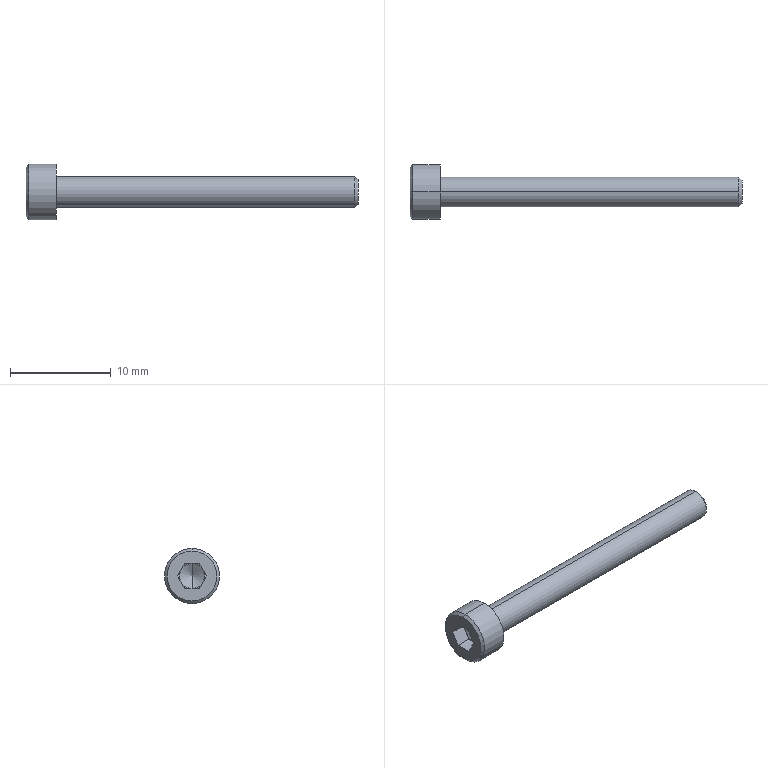Component | SolidWorks | TAC21-M3-L30Screw-1 | 1 solid | 25 faces | box 33 x 5.5 x 5.5 mm | volume 273 mm3 | plane 15 | cone 6 | cylinder 4 | commonest cylinder face diameters 3 x2 5.5 x2
STEP:
#1=COLOUR_RGB('',0.7922,0.8196,0.9333);
#2=FILL_AREA_STYLE_COLOUR('',#1);
#3=FILL_AREA_STYLE('',(#2));
#4=SURFACE_STYLE_FILL_AREA(#3);
#5=SURFACE_SIDE_STYLE('',(#4));
#6=SURFACE_STYLE_USAGE(.BOTH.,#5);
#7=PRESENTATION_STYLE_ASSIGNMENT((#6));
#8=CARTESIAN_POINT('',(-4.015,0.6298,4.665));
#9=VERTEX_POINT('',#8);
#10=CARTESIAN_POINT('',(-4.015,0.6298,4.547));
#11=VERTEX_POINT('',#10);
#12=CARTESIAN_POINT('',(-4.015,0.6298,4.606));
#13=DIRECTION('',(-1.,0.,0.));
#14=DIRECTION('',(0.,0.,1.));
#15=AXIS2_PLACEMENT_3D('',#12,#13,#14);
#16=CIRCLE('',#15,0.05906);
#17=EDGE_CURVE('',#9,#11,#16,.T.);
#18=ORIENTED_EDGE('',*,*,#17,.T.);
#19=CARTESIAN_POINT('',(-5.184,0.6298,4.547));
#20=VERTEX_POINT('',#19);
#21=CARTESIAN_POINT('',(-4.002,0.6298,4.547));
#22=DIRECTION('',(-1.,0.,0.));
#23=VECTOR('',#22,39.37);
#24=LINE('',#21,#23);
#25=EDGE_CURVE('',#11,#20,#24,.T.);
#26=ORIENTED_EDGE('',*,*,#25,.T.);
#27=CARTESIAN_POINT('',(-5.184,0.6298,4.665));
#28=VERTEX_POINT('',#27);
#29=CARTESIAN_POINT('',(-5.184,0.6298,4.606));
#30=DIRECTION('',(1.,0.,-0.));
#31=DIRECTION('',(0.,0.,1.));
#32=AXIS2_PLACEMENT_3D('',#29,#30,#31);
#33=CIRCLE('',#32,0.05906);
#34=EDGE_CURVE('',#20,#28,#33,.T.);
#35=ORIENTED_EDGE('',*,*,#34,.T.);
#36=CARTESIAN_POINT('',(-4.002,0.6298,4.665));
#37=DIRECTION('',(-1.,0.,0.));
#38=VECTOR('',#37,39.37);
#39=LINE('',#36,#38);
#40=EDGE_CURVE('',#9,#28,#39,.T.);
#41=ORIENTED_EDGE('',*,*,#40,.F.);
#42=EDGE_LOOP('',(#18,#26,#35,#41));
#43=FACE_OUTER_BOUND('',#42,.T.);
#44=CARTESIAN_POINT('',(-4.002,0.6298,4.606));
#45=DIRECTION('',(-1.,0.,0.));
#46=DIRECTION('',(0.,0.,1.));
#47=AXIS2_PLACEMENT_3D('',#44,#45,#46);
#48=CYLINDRICAL_SURFACE('',#47,0.05906);
#49=ADVANCED_FACE('',(#43),#48,.T.);
#50=CARTESIAN_POINT('',(-4.002,0.6298,4.653));
#51=VERTEX_POINT('',#50);
#52=CARTESIAN_POINT('',(-4.002,0.6298,4.559));
#53=VERTEX_POINT('',#52);
#54=CARTESIAN_POINT('',(-4.002,0.6298,4.606));
#55=DIRECTION('',(-1.,0.,0.));
#56=DIRECTION('',(0.,0.,1.));
#57=AXIS2_PLACEMENT_3D('',#54,#55,#56);
#58=CIRCLE('',#57,0.04699);
#59=EDGE_CURVE('',#51,#53,#58,.T.);
#60=ORIENTED_EDGE('',*,*,#59,.T.);
#61=CARTESIAN_POINT('',(-4.015,0.6298,4.547));
#62=DIRECTION('',(-0.7071,0.,-0.7071));
#63=VECTOR('',#62,39.37);
#64=LINE('',#61,#63);
#65=EDGE_CURVE('',#53,#11,#64,.T.);
#66=ORIENTED_EDGE('',*,*,#65,.T.);
#67=ORIENTED_EDGE('',*,*,#17,.F.);
#68=CARTESIAN_POINT('',(-4.015,0.6298,4.665));
#69=DIRECTION('',(-0.7071,0.,0.7071));
#70=VECTOR('',#69,39.37);
#71=LINE('',#68,#70);
#72=EDGE_CURVE('',#51,#9,#71,.T.);
#73=ORIENTED_EDGE('',*,*,#72,.F.);
#74=EDGE_LOOP('',(#60,#66,#67,#73));
#75=FACE_OUTER_BOUND('',#74,.T.);
#76=CARTESIAN_POINT('',(-4.015,0.6298,4.606));
#77=DIRECTION('',(-1.,0.,0.));
#78=DIRECTION('',(0.,0.,1.));
#79=AXIS2_PLACEMENT_3D('',#76,#77,#78);
#80=CONICAL_SURFACE('',#79,0.05906,0.7854);
#81=ADVANCED_FACE('',(#75),#80,.T.);
#82=CARTESIAN_POINT('',(-5.184,0.6298,4.715));
#83=VERTEX_POINT('',#82);
#84=CARTESIAN_POINT('',(-5.184,0.6298,4.498));
#85=VERTEX_POINT('',#84);
#86=CARTESIAN_POINT('',(-5.184,0.6298,4.606));
#87=DIRECTION('',(-1.,0.,0.));
#88=DIRECTION('',(0.,0.,1.));
#89=AXIS2_PLACEMENT_3D('',#86,#87,#88);
#90=CIRCLE('',#89,0.1083);
#91=EDGE_CURVE('',#83,#85,#90,.T.);
#92=ORIENTED_EDGE('',*,*,#91,.T.);
#93=CARTESIAN_POINT('',(-5.291,0.6298,4.498));
#94=VERTEX_POINT('',#93);
#95=CARTESIAN_POINT('',(-5.184,0.6298,4.498));
#96=DIRECTION('',(-1.,0.,0.));
#97=VECTOR('',#96,39.37);
#98=LINE('',#95,#97);
#99=EDGE_CURVE('',#85,#94,#98,.T.);
#100=ORIENTED_EDGE('',*,*,#99,.T.);
#101=CARTESIAN_POINT('',(-5.291,0.6298,4.715));
#102=VERTEX_POINT('',#101);
#103=CARTESIAN_POINT('',(-5.291,0.6298,4.606));
#104=DIRECTION('',(1.,0.,-0.));
#105=DIRECTION('',(0.,0.,1.));
#106=AXIS2_PLACEMENT_3D('',#103,#104,#105);
#107=CIRCLE('',#106,0.1083);
#108=EDGE_CURVE('',#94,#102,#107,.T.);
#109=ORIENTED_EDGE('',*,*,#108,.T.);
#110=CARTESIAN_POINT('',(-5.184,0.6298,4.715));
#111=DIRECTION('',(-1.,0.,0.));
#112=VECTOR('',#111,39.37);
#113=LINE('',#110,#112);
#114=EDGE_CURVE('',#83,#102,#113,.T.);
#115=ORIENTED_EDGE('',*,*,#114,.F.);
#116=EDGE_LOOP('',(#92,#100,#109,#115));
#117=FACE_OUTER_BOUND('',#116,.T.);
#118=CARTESIAN_POINT('',(-5.184,0.6298,4.606));
#119=DIRECTION('',(-1.,0.,0.));
#120=DIRECTION('',(0.,0.,1.));
#121=AXIS2_PLACEMENT_3D('',#118,#119,#120);
#122=CYLINDRICAL_SURFACE('',#121,0.1083);
#123=ADVANCED_FACE('',(#117),#122,.T.);
#124=CARTESIAN_POINT('',(-5.302,0.6298,4.509));
#125=VERTEX_POINT('',#124);
#126=CARTESIAN_POINT('',(-5.302,0.6298,4.704));
#127=VERTEX_POINT('',#126);
#128=CARTESIAN_POINT('',(-5.302,0.6298,4.606));
#129=DIRECTION('',(1.,0.,-0.));
#130=DIRECTION('',(0.,0.,-1.));
#131=AXIS2_PLACEMENT_3D('',#128,#129,#130);
#132=CIRCLE('',#131,0.09744);
#133=EDGE_CURVE('',#125,#127,#132,.T.);
#134=ORIENTED_EDGE('',*,*,#133,.T.);
#135=CARTESIAN_POINT('',(-5.291,0.6298,4.715));
#136=DIRECTION('',(0.7071,0.,0.7071));
#137=VECTOR('',#136,39.37);
#138=LINE('',#135,#137);
#139=EDGE_CURVE('',#127,#102,#138,.T.);
#140=ORIENTED_EDGE('',*,*,#139,.T.);
#141=ORIENTED_EDGE('',*,*,#108,.F.);
#142=CARTESIAN_POINT('',(-5.291,0.6298,4.498));
#143=DIRECTION('',(0.7071,0.,-0.7071));
#144=VECTOR('',#143,39.37);
#145=LINE('',#142,#144);
#146=EDGE_CURVE('',#125,#94,#145,.T.);
#147=ORIENTED_EDGE('',*,*,#146,.F.);
#148=EDGE_LOOP('',(#134,#140,#141,#147));
#149=FACE_OUTER_BOUND('',#148,.T.);
#150=CARTESIAN_POINT('',(-5.291,0.6298,4.606));
#151=DIRECTION('',(1.,0.,-0.));
#152=DIRECTION('',(0.,0.,-1.));
#153=AXIS2_PLACEMENT_3D('',#150,#151,#152);
#154=CONICAL_SURFACE('',#153,0.1083,0.7854);
#155=ADVANCED_FACE('',(#149),#154,.T.);
#156=CARTESIAN_POINT('',(-5.214,0.6298,4.606));
#157=VERTEX_POINT('',#156);
#158=CARTESIAN_POINT('',(-5.243,0.6298,4.656));
#159=VERTEX_POINT('',#158);
#160=CARTESIAN_POINT('',(-5.243,0.6298,4.656));
#161=DIRECTION('',(-0.5,0.,0.866));
#162=VECTOR('',#161,39.37);
#163=LINE('',#160,#162);
#164=EDGE_CURVE('',#157,#159,#163,.T.);
#165=ORIENTED_EDGE('',*,*,#164,.F.);
#166=CARTESIAN_POINT('',(-5.243,0.6298,4.557));
#167=VERTEX_POINT('',#166);
#168=CARTESIAN_POINT('',(-5.243,0.6298,4.557));
#169=DIRECTION('',(-0.5,0.,-0.866));
#170=VECTOR('',#169,39.37);
#171=LINE('',#168,#170);
#172=EDGE_CURVE('',#157,#167,#171,.T.);
#173=ORIENTED_EDGE('',*,*,#172,.T.);
#174=CARTESIAN_POINT('',(-5.243,0.5871,4.582));
#175=VERTEX_POINT('',#174);
#176=CARTESIAN_POINT('',(-5.243,0.6298,4.606));
#177=DIRECTION('',(1.,0.,-0.));
#178=DIRECTION('',(0.,0.,1.));
#179=AXIS2_PLACEMENT_3D('',#176,#177,#178);
#180=CIRCLE('',#179,0.04921);
#181=EDGE_CURVE('',#175,#167,#180,.T.);
#182=ORIENTED_EDGE('',*,*,#181,.F.);
#183=CARTESIAN_POINT('',(-5.243,0.5871,4.631));
#184=VERTEX_POINT('',#183);
#185=CARTESIAN_POINT('',(-5.243,0.6298,4.606));
#186=DIRECTION('',(1.,0.,-0.));
#187=DIRECTION('',(0.,-0.,1.));
#188=AXIS2_PLACEMENT_3D('',#185,#186,#187);
#189=CIRCLE('',#188,0.04921);
#190=EDGE_CURVE('',#184,#175,#189,.T.);
#191=ORIENTED_EDGE('',*,*,#190,.F.);
#192=CARTESIAN_POINT('',(-5.243,0.6298,4.606));
#193=DIRECTION('',(1.,0.,-0.));
#194=DIRECTION('',(0.,0.,1.));
#195=AXIS2_PLACEMENT_3D('',#192,#193,#194);
#196=CIRCLE('',#195,0.04921);
#197=EDGE_CURVE('',#159,#184,#196,.T.);
#198=ORIENTED_EDGE('',*,*,#197,.F.);
#199=EDGE_LOOP('',(#165,#173,#182,#191,#198));
#200=FACE_OUTER_BOUND('',#199,.T.);
#201=CARTESIAN_POINT('',(-5.243,0.6298,4.606));
#202=DIRECTION('',(-1.,0.,0.));
#203=DIRECTION('',(0.,0.,1.));
#204=AXIS2_PLACEMENT_3D('',#201,#202,#203);
#205=CONICAL_SURFACE('',#204,0.04921,1.047);
#206=ADVANCED_FACE('',(#200),#205,.F.);
#207=ORIENTED_EDGE('',*,*,#25,.F.);
#208=CARTESIAN_POINT('',(-4.015,0.6298,4.606));
#209=DIRECTION('',(-1.,0.,0.));
#210=DIRECTION('',(0.,0.,1.));
#211=AXIS2_PLACEMENT_3D('',#208,#209,#210);
#212=CIRCLE('',#211,0.05906);
#213=EDGE_CURVE('',#11,#9,#212,.T.);
#214=ORIENTED_EDGE('',*,*,#213,.T.);
#215=ORIENTED_EDGE('',*,*,#40,.T.);
#216=CARTESIAN_POINT('',(-5.184,0.6298,4.606));
#217=DIRECTION('',(1.,0.,-0.));
#218=DIRECTION('',(0.,0.,1.));
#219=AXIS2_PLACEMENT_3D('',#216,#217,#218);
#220=CIRCLE('',#219,0.05906);
#221=EDGE_CURVE('',#28,#20,#220,.T.);
#222=ORIENTED_EDGE('',*,*,#221,.T.);
#223=EDGE_LOOP('',(#207,#214,#215,#222));
#224=FACE_OUTER_BOUND('',#223,.T.);
#225=CARTESIAN_POINT('',(-4.002,0.6298,4.606));
#226=DIRECTION('',(-1.,0.,0.));
#227=DIRECTION('',(0.,0.,1.));
#228=AXIS2_PLACEMENT_3D('',#225,#226,#227);
#229=CYLINDRICAL_SURFACE('',#228,0.05906);
#230=ADVANCED_FACE('',(#224),#229,.T.);
#231=ORIENTED_EDGE('',*,*,#91,.F.);
#232=CARTESIAN_POINT('',(-5.184,0.6298,4.606));
#233=DIRECTION('',(-1.,0.,0.));
#234=DIRECTION('',(0.,0.,1.));
#235=AXIS2_PLACEMENT_3D('',#232,#233,#234);
#236=CIRCLE('',#235,0.1083);
#237=EDGE_CURVE('',#85,#83,#236,.T.);
#238=ORIENTED_EDGE('',*,*,#237,.F.);
#239=EDGE_LOOP('',(#231,#238));
#240=FACE_OUTER_BOUND('',#239,.T.);
#241=ORIENTED_EDGE('',*,*,#221,.F.);
#242=ORIENTED_EDGE('',*,*,#34,.F.);
#243=EDGE_LOOP('',(#241,#242));
#244=FACE_BOUND('',#243,.T.);
#245=CARTESIAN_POINT('',(-5.184,0.738,4.606));
#246=DIRECTION('',(-1.,0.,0.));
#247=DIRECTION('',(0.,0.,1.));
#248=AXIS2_PLACEMENT_3D('',#245,#246,#247);
#249=PLANE('',#248);
#250=ADVANCED_FACE('',(#240,#244),#249,.F.);
#251=ORIENTED_EDGE('',*,*,#65,.F.);
#252=CARTESIAN_POINT('',(-4.002,0.6298,4.606));
#253=DIRECTION('',(-1.,0.,0.));
#254=DIRECTION('',(0.,0.,1.));
#255=AXIS2_PLACEMENT_3D('',#252,#253,#254);
#256=CIRCLE('',#255,0.04699);
#257=EDGE_CURVE('',#53,#51,#256,.T.);
#258=ORIENTED_EDGE('',*,*,#257,.T.);
#259=ORIENTED_EDGE('',*,*,#72,.T.);
#260=ORIENTED_EDGE('',*,*,#213,.F.);
#261=EDGE_LOOP('',(#251,#258,#259,#260));
#262=FACE_OUTER_BOUND('',#261,.T.);
#263=CARTESIAN_POINT('',(-4.015,0.6298,4.606));
#264=DIRECTION('',(-1.,0.,0.));
#265=DIRECTION('',(0.,0.,1.));
#266=AXIS2_PLACEMENT_3D('',#263,#264,#265);
#267=CONICAL_SURFACE('',#266,0.05906,0.7854);
#268=ADVANCED_FACE('',(#262),#267,.T.);
#269=ORIENTED_EDGE('',*,*,#99,.F.);
#270=ORIENTED_EDGE('',*,*,#237,.T.);
#271=ORIENTED_EDGE('',*,*,#114,.T.);
#272=CARTESIAN_POINT('',(-5.291,0.6298,4.606));
#273=DIRECTION('',(1.,0.,-0.));
#274=DIRECTION('',(0.,0.,1.));
#275=AXIS2_PLACEMENT_3D('',#272,#273,#274);
#276=CIRCLE('',#275,0.1083);
#277=EDGE_CURVE('',#102,#94,#276,.T.);
#278=ORIENTED_EDGE('',*,*,#277,.T.);
#279=EDGE_LOOP('',(#269,#270,#271,#278));
#280=FACE_OUTER_BOUND('',#279,.T.);
#281=CARTESIAN_POINT('',(-5.184,0.6298,4.606));
#282=DIRECTION('',(-1.,0.,0.));
#283=DIRECTION('',(0.,0.,1.));
#284=AXIS2_PLACEMENT_3D('',#281,#282,#283);
#285=CYLINDRICAL_SURFACE('',#284,0.1083);
#286=ADVANCED_FACE('',(#280),#285,.T.);
#287=ORIENTED_EDGE('',*,*,#59,.F.);
#288=ORIENTED_EDGE('',*,*,#257,.F.);
#289=EDGE_LOOP('',(#287,#288));
#290=FACE_OUTER_BOUND('',#289,.T.);
#291=CARTESIAN_POINT('',(-4.002,0.6767,4.606));
#292=DIRECTION('',(-1.,0.,0.));
#293=DIRECTION('',(0.,0.,1.));
#294=AXIS2_PLACEMENT_3D('',#291,#292,#293);
#295=PLANE('',#294);
#296=ADVANCED_FACE('',(#290),#295,.F.);
#297=ORIENTED_EDGE('',*,*,#139,.F.);
#298=CARTESIAN_POINT('',(-5.302,0.6298,4.606));
#299=DIRECTION('',(1.,0.,-0.));
#300=DIRECTION('',(0.,0.,-1.));
#301=AXIS2_PLACEMENT_3D('',#298,#299,#300);
#302=CIRCLE('',#301,0.09744);
#303=EDGE_CURVE('',#127,#125,#302,.T.);
#304=ORIENTED_EDGE('',*,*,#303,.T.);
#305=ORIENTED_EDGE('',*,*,#146,.T.);
#306=ORIENTED_EDGE('',*,*,#277,.F.);
#307=EDGE_LOOP('',(#297,#304,#305,#306));
#308=FACE_OUTER_BOUND('',#307,.T.);
#309=CARTESIAN_POINT('',(-5.291,0.6298,4.606));
#310=DIRECTION('',(1.,0.,-0.));
#311=DIRECTION('',(0.,0.,-1.));
#312=AXIS2_PLACEMENT_3D('',#309,#310,#311);
#313=CONICAL_SURFACE('',#312,0.1083,0.7854);
#314=ADVANCED_FACE('',(#308),#313,.T.);
#315=CARTESIAN_POINT('',(-5.302,0.6013,4.557));
#316=VERTEX_POINT('',#315);
#317=CARTESIAN_POINT('',(-5.302,0.5729,4.606));
#318=VERTEX_POINT('',#317);
#319=CARTESIAN_POINT('',(-5.302,0.6013,4.557));
#320=DIRECTION('',(0.,-0.5,0.866));
#321=VECTOR('',#320,39.37);
#322=LINE('',#319,#321);
#323=EDGE_CURVE('',#316,#318,#322,.T.);
#324=ORIENTED_EDGE('',*,*,#323,.F.);
#325=CARTESIAN_POINT('',(-5.302,0.6582,4.557));
#326=VERTEX_POINT('',#325);
#327=CARTESIAN_POINT('',(-5.302,0.6298,4.557));
#328=DIRECTION('',(0.,-1.,0.));
#329=VECTOR('',#328,39.37);
#330=LINE('',#327,#329);
#331=EDGE_CURVE('',#326,#316,#330,.T.);
#332=ORIENTED_EDGE('',*,*,#331,.F.);
#333=CARTESIAN_POINT('',(-5.302,0.6866,4.606));
#334=VERTEX_POINT('',#333);
#335=CARTESIAN_POINT('',(-5.302,0.6866,4.606));
#336=DIRECTION('',(-0.,-0.5,-0.866));
#337=VECTOR('',#336,39.37);
#338=LINE('',#335,#337);
#339=EDGE_CURVE('',#334,#326,#338,.T.);
#340=ORIENTED_EDGE('',*,*,#339,.F.);
#341=CARTESIAN_POINT('',(-5.302,0.6582,4.656));
#342=VERTEX_POINT('',#341);
#343=CARTESIAN_POINT('',(-5.302,0.6582,4.656));
#344=DIRECTION('',(-0.,0.5,-0.866));
#345=VECTOR('',#344,39.37);
#346=LINE('',#343,#345);
#347=EDGE_CURVE('',#342,#334,#346,.T.);
#348=ORIENTED_EDGE('',*,*,#347,.F.);
#349=CARTESIAN_POINT('',(-5.302,0.6013,4.656));
#350=VERTEX_POINT('',#349);
#351=CARTESIAN_POINT('',(-5.302,0.6298,4.656));
#352=DIRECTION('',(0.,1.,0.));
#353=VECTOR('',#352,39.37);
#354=LINE('',#351,#353);
#355=EDGE_CURVE('',#350,#342,#354,.T.);
#356=ORIENTED_EDGE('',*,*,#355,.F.);
#357=CARTESIAN_POINT('',(-5.302,0.5729,4.606));
#358=DIRECTION('',(0.,0.5,0.866));
#359=VECTOR('',#358,39.37);
#360=LINE('',#357,#359);
#361=EDGE_CURVE('',#318,#350,#360,.T.);
#362=ORIENTED_EDGE('',*,*,#361,.F.);
#363=EDGE_LOOP('',(#324,#332,#340,#348,#356,#362));
#364=FACE_BOUND('',#363,.T.);
#365=ORIENTED_EDGE('',*,*,#133,.F.);
#366=ORIENTED_EDGE('',*,*,#303,.F.);
#367=EDGE_LOOP('',(#365,#366));
#368=FACE_OUTER_BOUND('',#367,.T.);
#369=CARTESIAN_POINT('',(-5.302,0.6298,4.606));
#370=DIRECTION('',(1.,0.,-0.));
#371=DIRECTION('',(-0.,0.,-1.));
#372=AXIS2_PLACEMENT_3D('',#369,#370,#371);
#373=PLANE('',#372);
#374=ADVANCED_FACE('',(#364,#368),#373,.F.);
#375=CARTESIAN_POINT('',(-5.243,0.6013,4.656));
#376=VERTEX_POINT('',#375);
#377=CARTESIAN_POINT('',(-5.243,0.6013,4.656));
#378=DIRECTION('',(-1.,0.,0.));
#379=VECTOR('',#378,39.37);
#380=LINE('',#377,#379);
#381=EDGE_CURVE('',#376,#350,#380,.T.);
#382=ORIENTED_EDGE('',*,*,#381,.F.);
#383=CARTESIAN_POINT('',(-5.243,0.5729,4.606));
#384=DIRECTION('',(0.,0.5,0.866));
#385=VECTOR('',#384,39.37);
#386=LINE('',#383,#385);
#387=EDGE_CURVE('',#184,#376,#386,.T.);
#388=ORIENTED_EDGE('',*,*,#387,.F.);
#389=CARTESIAN_POINT('',(-5.243,0.5729,4.606));
#390=VERTEX_POINT('',#389);
#391=CARTESIAN_POINT('',(-5.243,0.5729,4.606));
#392=DIRECTION('',(0.,0.5,0.866));
#393=VECTOR('',#392,39.37);
#394=LINE('',#391,#393);
#395=EDGE_CURVE('',#390,#184,#394,.T.);
#396=ORIENTED_EDGE('',*,*,#395,.F.);
#397=CARTESIAN_POINT('',(-5.243,0.5729,4.606));
#398=DIRECTION('',(1.,0.,-0.));
#399=VECTOR('',#398,39.37);
#400=LINE('',#397,#399);
#401=EDGE_CURVE('',#318,#390,#400,.T.);
#402=ORIENTED_EDGE('',*,*,#401,.F.);
#403=ORIENTED_EDGE('',*,*,#361,.T.);
#404=EDGE_LOOP('',(#382,#388,#396,#402,#403));
#405=FACE_OUTER_BOUND('',#404,.T.);
#406=CARTESIAN_POINT('',(-5.243,0.5729,4.606));
#407=DIRECTION('',(0.,-0.866,0.5));
#408=DIRECTION('',(0.,0.5,0.866));
#409=AXIS2_PLACEMENT_3D('',#406,#407,#408);
#410=PLANE('',#409);
#411=ADVANCED_FACE('',(#405),#410,.F.);
#412=ORIENTED_EDGE('',*,*,#401,.T.);
#413=CARTESIAN_POINT('',(-5.243,0.6013,4.557));
#414=DIRECTION('',(0.,-0.5,0.866));
#415=VECTOR('',#414,39.37);
#416=LINE('',#413,#415);
#417=EDGE_CURVE('',#175,#390,#416,.T.);
#418=ORIENTED_EDGE('',*,*,#417,.F.);
#419=CARTESIAN_POINT('',(-5.243,0.6013,4.557));
#420=VERTEX_POINT('',#419);
#421=CARTESIAN_POINT('',(-5.243,0.6013,4.557));
#422=DIRECTION('',(0.,-0.5,0.866));
#423=VECTOR('',#422,39.37);
#424=LINE('',#421,#423);
#425=EDGE_CURVE('',#420,#175,#424,.T.);
#426=ORIENTED_EDGE('',*,*,#425,.F.);
#427=CARTESIAN_POINT('',(-5.243,0.6013,4.557));
#428=DIRECTION('',(1.,0.,-0.));
#429=VECTOR('',#428,39.37);
#430=LINE('',#427,#429);
#431=EDGE_CURVE('',#316,#420,#430,.T.);
#432=ORIENTED_EDGE('',*,*,#431,.F.);
#433=ORIENTED_EDGE('',*,*,#323,.T.);
#434=EDGE_LOOP('',(#412,#418,#426,#432,#433));
#435=FACE_OUTER_BOUND('',#434,.T.);
#436=CARTESIAN_POINT('',(-5.243,0.6013,4.557));
#437=DIRECTION('',(-0.,-0.866,-0.5));
#438=DIRECTION('',(0.,-0.5,0.866));
#439=AXIS2_PLACEMENT_3D('',#436,#437,#438);
#440=PLANE('',#439);
#441=ADVANCED_FACE('',(#435),#440,.F.);
#442=ORIENTED_EDGE('',*,*,#431,.T.);
#443=CARTESIAN_POINT('',(-5.243,0.6582,4.557));
#444=DIRECTION('',(0.,-1.,0.));
#445=VECTOR('',#444,39.37);
#446=LINE('',#443,#445);
#447=EDGE_CURVE('',#167,#420,#446,.T.);
#448=ORIENTED_EDGE('',*,*,#447,.F.);
#449=CARTESIAN_POINT('',(-5.243,0.6582,4.557));
#450=VERTEX_POINT('',#449);
#451=CARTESIAN_POINT('',(-5.243,0.6582,4.557));
#452=DIRECTION('',(0.,-1.,0.));
#453=VECTOR('',#452,39.37);
#454=LINE('',#451,#453);
#455=EDGE_CURVE('',#450,#167,#454,.T.);
#456=ORIENTED_EDGE('',*,*,#455,.F.);
#457=CARTESIAN_POINT('',(-5.243,0.6582,4.557));
#458=DIRECTION('',(1.,0.,-0.));
#459=VECTOR('',#458,39.37);
#460=LINE('',#457,#459);
#461=EDGE_CURVE('',#326,#450,#460,.T.);
#462=ORIENTED_EDGE('',*,*,#461,.F.);
#463=ORIENTED_EDGE('',*,*,#331,.T.);
#464=EDGE_LOOP('',(#442,#448,#456,#462,#463));
#465=FACE_OUTER_BOUND('',#464,.T.);
#466=CARTESIAN_POINT('',(-5.243,0.6582,4.557));
#467=DIRECTION('',(-0.,0.,-1.));
#468=DIRECTION('',(-1.,0.,0.));
#469=AXIS2_PLACEMENT_3D('',#466,#467,#468);
#470=PLANE('',#469);
#471=ADVANCED_FACE('',(#465),#470,.F.);
#472=ORIENTED_EDGE('',*,*,#461,.T.);
#473=CARTESIAN_POINT('',(-5.243,0.6724,4.582));
#474=VERTEX_POINT('',#473);
#475=CARTESIAN_POINT('',(-5.243,0.6866,4.606));
#476=DIRECTION('',(-0.,-0.5,-0.866));
#477=VECTOR('',#476,39.37);
#478=LINE('',#475,#477);
#479=EDGE_CURVE('',#474,#450,#478,.T.);
#480=ORIENTED_EDGE('',*,*,#479,.F.);
#481=CARTESIAN_POINT('',(-5.243,0.6866,4.606));
#482=VERTEX_POINT('',#481);
#483=CARTESIAN_POINT('',(-5.243,0.6866,4.606));
#484=DIRECTION('',(-0.,-0.5,-0.866));
#485=VECTOR('',#484,39.37);
#486=LINE('',#483,#485);
#487=EDGE_CURVE('',#482,#474,#486,.T.);
#488=ORIENTED_EDGE('',*,*,#487,.F.);
#489=CARTESIAN_POINT('',(-5.243,0.6866,4.606));
#490=DIRECTION('',(1.,0.,-0.));
#491=VECTOR('',#490,39.37);
#492=LINE('',#489,#491);
#493=EDGE_CURVE('',#334,#482,#492,.T.);
#494=ORIENTED_EDGE('',*,*,#493,.F.);
#495=ORIENTED_EDGE('',*,*,#339,.T.);
#496=EDGE_LOOP('',(#472,#480,#488,#494,#495));
#497=FACE_OUTER_BOUND('',#496,.T.);
#498=CARTESIAN_POINT('',(-5.243,0.6866,4.606));
#499=DIRECTION('',(-0.,0.866,-0.5));
#500=DIRECTION('',(-0.,-0.5,-0.866));
#501=AXIS2_PLACEMENT_3D('',#498,#499,#500);
#502=PLANE('',#501);
#503=ADVANCED_FACE('',(#497),#502,.F.);
#504=ORIENTED_EDGE('',*,*,#493,.T.);
#505=CARTESIAN_POINT('',(-5.243,0.6724,4.631));
#506=VERTEX_POINT('',#505);
#507=CARTESIAN_POINT('',(-5.243,0.6582,4.656));
#508=DIRECTION('',(-0.,0.5,-0.866));
#509=VECTOR('',#508,39.37);
#510=LINE('',#507,#509);
#511=EDGE_CURVE('',#506,#482,#510,.T.);
#512=ORIENTED_EDGE('',*,*,#511,.F.);
#513=CARTESIAN_POINT('',(-5.243,0.6582,4.656));
#514=VERTEX_POINT('',#513);
#515=CARTESIAN_POINT('',(-5.243,0.6582,4.656));
#516=DIRECTION('',(-0.,0.5,-0.866));
#517=VECTOR('',#516,39.37);
#518=LINE('',#515,#517);
#519=EDGE_CURVE('',#514,#506,#518,.T.);
#520=ORIENTED_EDGE('',*,*,#519,.F.);
#521=CARTESIAN_POINT('',(-5.243,0.6582,4.656));
#522=DIRECTION('',(1.,0.,-0.));
#523=VECTOR('',#522,39.37);
#524=LINE('',#521,#523);
#525=EDGE_CURVE('',#342,#514,#524,.T.);
#526=ORIENTED_EDGE('',*,*,#525,.F.);
#527=ORIENTED_EDGE('',*,*,#347,.T.);
#528=EDGE_LOOP('',(#504,#512,#520,#526,#527));
#529=FACE_OUTER_BOUND('',#528,.T.);
#530=CARTESIAN_POINT('',(-5.243,0.6582,4.656));
#531=DIRECTION('',(0.,0.866,0.5));
#532=DIRECTION('',(-0.,0.5,-0.866));
#533=AXIS2_PLACEMENT_3D('',#530,#531,#532);
#534=PLANE('',#533);
#535=ADVANCED_FACE('',(#529),#534,.F.);
#536=ORIENTED_EDGE('',*,*,#525,.T.);
#537=CARTESIAN_POINT('',(-5.243,0.6013,4.656));
#538=DIRECTION('',(0.,1.,0.));
#539=VECTOR('',#538,39.37);
#540=LINE('',#537,#539);
#541=EDGE_CURVE('',#159,#514,#540,.T.);
#542=ORIENTED_EDGE('',*,*,#541,.F.);
#543=CARTESIAN_POINT('',(-5.243,0.6013,4.656));
#544=DIRECTION('',(0.,1.,0.));
#545=VECTOR('',#544,39.37);
#546=LINE('',#543,#545);
#547=EDGE_CURVE('',#376,#159,#546,.T.);
#548=ORIENTED_EDGE('',*,*,#547,.F.);
#549=ORIENTED_EDGE('',*,*,#381,.T.);
#550=ORIENTED_EDGE('',*,*,#355,.T.);
#551=EDGE_LOOP('',(#536,#542,#548,#549,#550));
#552=FACE_OUTER_BOUND('',#551,.T.);
#553=CARTESIAN_POINT('',(-5.243,0.6013,4.656));
#554=DIRECTION('',(0.,0.,1.));
#555=DIRECTION('',(1.,0.,-0.));
#556=AXIS2_PLACEMENT_3D('',#553,#554,#555);
#557=PLANE('',#556);
#558=ADVANCED_FACE('',(#552),#557,.F.);
#559=ORIENTED_EDGE('',*,*,#197,.T.);
#560=ORIENTED_EDGE('',*,*,#387,.T.);
#561=ORIENTED_EDGE('',*,*,#547,.T.);
#562=EDGE_LOOP('',(#559,#560,#561));
#563=FACE_OUTER_BOUND('',#562,.T.);
#564=CARTESIAN_POINT('',(-5.243,0.6298,4.606));
#565=DIRECTION('',(-1.,0.,0.));
#566=DIRECTION('',(0.,0.,1.));
#567=AXIS2_PLACEMENT_3D('',#564,#565,#566);
#568=PLANE('',#567);
#569=ADVANCED_FACE('',(#563),#568,.T.);
#570=ORIENTED_EDGE('',*,*,#190,.T.);
#571=ORIENTED_EDGE('',*,*,#417,.T.);
#572=ORIENTED_EDGE('',*,*,#395,.T.);
#573=EDGE_LOOP('',(#570,#571,#572));
#574=FACE_OUTER_BOUND('',#573,.T.);
#575=CARTESIAN_POINT('',(-5.243,0.6298,4.606));
#576=DIRECTION('',(-1.,0.,0.));
#577=DIRECTION('',(0.,0.,1.));
#578=AXIS2_PLACEMENT_3D('',#575,#576,#577);
#579=PLANE('',#578);
#580=ADVANCED_FACE('',(#574),#579,.T.);
#581=ORIENTED_EDGE('',*,*,#181,.T.);
#582=ORIENTED_EDGE('',*,*,#447,.T.);
#583=ORIENTED_EDGE('',*,*,#425,.T.);
#584=EDGE_LOOP('',(#581,#582,#583));
#585=FACE_OUTER_BOUND('',#584,.T.);
#586=CARTESIAN_POINT('',(-5.243,0.6298,4.606));
#587=DIRECTION('',(-1.,0.,0.));
#588=DIRECTION('',(0.,0.,1.));
#589=AXIS2_PLACEMENT_3D('',#586,#587,#588);
#590=PLANE('',#589);
#591=ADVANCED_FACE('',(#585),#590,.T.);
#592=CARTESIAN_POINT('',(-5.243,0.6298,4.606));
#593=DIRECTION('',(1.,0.,-0.));
#594=DIRECTION('',(0.,0.,1.));
#595=AXIS2_PLACEMENT_3D('',#592,#593,#594);
#596=CIRCLE('',#595,0.04921);
#597=EDGE_CURVE('',#167,#474,#596,.T.);
#598=ORIENTED_EDGE('',*,*,#597,.T.);
#599=ORIENTED_EDGE('',*,*,#479,.T.);
#600=ORIENTED_EDGE('',*,*,#455,.T.);
#601=EDGE_LOOP('',(#598,#599,#600));
#602=FACE_OUTER_BOUND('',#601,.T.);
#603=CARTESIAN_POINT('',(-5.243,0.6298,4.606));
#604=DIRECTION('',(-1.,0.,0.));
#605=DIRECTION('',(0.,0.,1.));
#606=AXIS2_PLACEMENT_3D('',#603,#604,#605);
#607=PLANE('',#606);
#608=ADVANCED_FACE('',(#602),#607,.T.);
#609=CARTESIAN_POINT('',(-5.243,0.6298,4.606));
#610=DIRECTION('',(1.,0.,-0.));
#611=DIRECTION('',(0.,-0.,1.));
#612=AXIS2_PLACEMENT_3D('',#609,#610,#611);
#613=CIRCLE('',#612,0.04921);
#614=EDGE_CURVE('',#474,#506,#613,.T.);
#615=ORIENTED_EDGE('',*,*,#614,.T.);
#616=ORIENTED_EDGE('',*,*,#511,.T.);
#617=ORIENTED_EDGE('',*,*,#487,.T.);
#618=EDGE_LOOP('',(#615,#616,#617));
#619=FACE_OUTER_BOUND('',#618,.T.);
#620=CARTESIAN_POINT('',(-5.243,0.6298,4.606));
#621=DIRECTION('',(-1.,0.,0.));
#622=DIRECTION('',(0.,0.,1.));
#623=AXIS2_PLACEMENT_3D('',#620,#621,#622);
#624=PLANE('',#623);
#625=ADVANCED_FACE('',(#619),#624,.T.);
#626=CARTESIAN_POINT('',(-5.243,0.6298,4.606));
#627=DIRECTION('',(1.,0.,-0.));
#628=DIRECTION('',(0.,0.,1.));
#629=AXIS2_PLACEMENT_3D('',#626,#627,#628);
#630=CIRCLE('',#629,0.04921);
#631=EDGE_CURVE('',#506,#159,#630,.T.);
#632=ORIENTED_EDGE('',*,*,#631,.T.);
#633=ORIENTED_EDGE('',*,*,#541,.T.);
#634=ORIENTED_EDGE('',*,*,#519,.T.);
#635=EDGE_LOOP('',(#632,#633,#634));
#636=FACE_OUTER_BOUND('',#635,.T.);
#637=CARTESIAN_POINT('',(-5.243,0.6298,4.606));
#638=DIRECTION('',(-1.,0.,0.));
#639=DIRECTION('',(0.,0.,1.));
#640=AXIS2_PLACEMENT_3D('',#637,#638,#639);
#641=PLANE('',#640);
#642=ADVANCED_FACE('',(#636),#641,.T.);
#643=ORIENTED_EDGE('',*,*,#172,.F.);
#644=ORIENTED_EDGE('',*,*,#164,.T.);
#645=ORIENTED_EDGE('',*,*,#631,.F.);
#646=ORIENTED_EDGE('',*,*,#614,.F.);
#647=ORIENTED_EDGE('',*,*,#597,.F.);
#648=EDGE_LOOP('',(#643,#644,#645,#646,#647));
#649=FACE_OUTER_BOUND('',#648,.T.);
#650=CARTESIAN_POINT('',(-5.243,0.6298,4.606));
#651=DIRECTION('',(-1.,0.,0.));
#652=DIRECTION('',(0.,0.,1.));
#653=AXIS2_PLACEMENT_3D('',#650,#651,#652);
#654=CONICAL_SURFACE('',#653,0.04921,1.047);
#655=ADVANCED_FACE('',(#649),#654,.F.);
#656=CLOSED_SHELL('',(#49,#81,#123,#155,#206,#230,#250,#268,#286,#296,#314,#374,#411,#441,#471,#503,#535,#558,#569,#580,#591,#608,#625,#642,#655));
#657=MANIFOLD_SOLID_BREP('',#656);
#658=STYLED_ITEM('',(#7),#657);
#659=PRESENTATION_LAYER_ASSIGNMENT('','',(#658));
#660=(LENGTH_UNIT()NAMED_UNIT(*)SI_UNIT($,.METRE.));
#661=LENGTH_MEASURE_WITH_UNIT(LENGTH_MEASURE(0.0254),#660);
#662=DIMENSIONAL_EXPONENTS(1.,0.,0.,0.,0.,0.,0.);
#663=(CONVERSION_BASED_UNIT('',#661)LENGTH_UNIT()NAMED_UNIT(#662));
#664=UNCERTAINTY_MEASURE_WITH_UNIT(LENGTH_MEASURE(0.00001),#663,'','');
#665=(NAMED_UNIT(*)PLANE_ANGLE_UNIT()SI_UNIT($,.RADIAN.));
#666=(NAMED_UNIT(*)SI_UNIT($,.STERADIAN.)SOLID_ANGLE_UNIT());
#667=(GEOMETRIC_REPRESENTATION_CONTEXT(3)GLOBAL_UNCERTAINTY_ASSIGNED_CONTEXT((#664))GLOBAL_UNIT_ASSIGNED_CONTEXT((#663,#665,#666))REPRESENTATION_CONTEXT('',''));
#668=MECHANICAL_DESIGN_GEOMETRIC_PRESENTATION_REPRESENTATION('',(#658),#667);
#669=CARTESIAN_POINT('',(0.,0.,0.));
#670=DIRECTION('',(0.,0.,1.));
#671=DIRECTION('',(1.,0.,0.));
#672=AXIS2_PLACEMENT_3D('',#669,#670,#671);
#673=(LENGTH_UNIT()NAMED_UNIT(*)SI_UNIT($,.METRE.));
#674=LENGTH_MEASURE_WITH_UNIT(LENGTH_MEASURE(0.0254),#673);
#675=DIMENSIONAL_EXPONENTS(1.,0.,0.,0.,0.,0.,0.);
#676=(CONVERSION_BASED_UNIT('',#674)LENGTH_UNIT()NAMED_UNIT(#675));
#677=UNCERTAINTY_MEASURE_WITH_UNIT(LENGTH_MEASURE(0.00001),#676,'','');
#678=(NAMED_UNIT(*)PLANE_ANGLE_UNIT()SI_UNIT($,.RADIAN.));
#679=(NAMED_UNIT(*)SI_UNIT($,.STERADIAN.)SOLID_ANGLE_UNIT());
#680=(GEOMETRIC_REPRESENTATION_CONTEXT(3)GLOBAL_UNCERTAINTY_ASSIGNED_CONTEXT((#677))GLOBAL_UNIT_ASSIGNED_CONTEXT((#676,#678,#679))REPRESENTATION_CONTEXT('',''));
#681=ADVANCED_BREP_SHAPE_REPRESENTATION('',(#657,#672),#680);